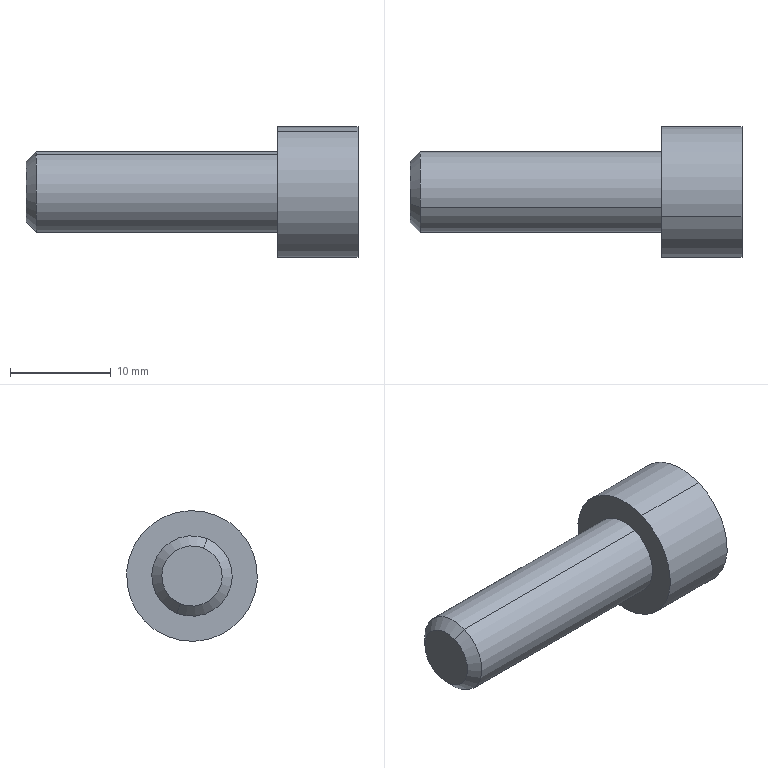Component | SolidWorks | 10HexSocketScrewM8X25-2 | 1 solid | 23 faces | box 33 x 13 x 13 mm | volume 2111 mm3 | plane 15 | cone 4 | cylinder 4 | commonest cylinder face diameters 8 x2 13 x2
STEP:
#1=COLOUR_RGB('',0.7922,0.8196,0.9333);
#2=FILL_AREA_STYLE_COLOUR('',#1);
#3=FILL_AREA_STYLE('',(#2));
#4=SURFACE_STYLE_FILL_AREA(#3);
#5=SURFACE_SIDE_STYLE('',(#4));
#6=SURFACE_STYLE_USAGE(.BOTH.,#5);
#7=PRESENTATION_STYLE_ASSIGNMENT((#6));
#8=CARTESIAN_POINT('',(3.66,-0.8593,8.759));
#9=VERTEX_POINT('',#8);
#10=CARTESIAN_POINT('',(3.66,-0.9495,8.977));
#11=VERTEX_POINT('',#10);
#12=CARTESIAN_POINT('',(3.66,-0.9044,8.868));
#13=DIRECTION('',(-1.,-0.,-0.));
#14=DIRECTION('',(0.,0.3818,-0.9242));
#15=AXIS2_PLACEMENT_3D('',#12,#13,#14);
#16=CIRCLE('',#15,0.1181);
#17=EDGE_CURVE('',#9,#11,#16,.T.);
#18=ORIENTED_EDGE('',*,*,#17,.F.);
#19=CARTESIAN_POINT('',(3.699,-0.8443,8.723));
#20=VERTEX_POINT('',#19);
#21=CARTESIAN_POINT('',(3.66,-0.8593,8.759));
#22=DIRECTION('',(0.7071,0.27,-0.6535));
#23=VECTOR('',#22,39.37);
#24=LINE('',#21,#23);
#25=EDGE_CURVE('',#9,#20,#24,.T.);
#26=ORIENTED_EDGE('',*,*,#25,.T.);
#27=CARTESIAN_POINT('',(3.699,-0.9646,9.014));
#28=VERTEX_POINT('',#27);
#29=CARTESIAN_POINT('',(3.699,-0.9044,8.868));
#30=DIRECTION('',(1.,0.,0.));
#31=DIRECTION('',(0.,0.3818,-0.9242));
#32=AXIS2_PLACEMENT_3D('',#29,#30,#31);
#33=CIRCLE('',#32,0.1575);
#34=EDGE_CURVE('',#28,#20,#33,.T.);
#35=ORIENTED_EDGE('',*,*,#34,.F.);
#36=CARTESIAN_POINT('',(3.66,-0.9495,8.977));
#37=DIRECTION('',(0.7071,-0.27,0.6535));
#38=VECTOR('',#37,39.37);
#39=LINE('',#36,#38);
#40=EDGE_CURVE('',#11,#28,#39,.T.);
#41=ORIENTED_EDGE('',*,*,#40,.F.);
#42=EDGE_LOOP('',(#18,#26,#35,#41));
#43=FACE_OUTER_BOUND('',#42,.T.);
#44=CARTESIAN_POINT('',(3.66,-0.9044,8.868));
#45=DIRECTION('',(1.,0.,0.));
#46=DIRECTION('',(0.,-0.3818,0.9242));
#47=AXIS2_PLACEMENT_3D('',#44,#45,#46);
#48=CONICAL_SURFACE('',#47,0.1181,0.7854);
#49=ADVANCED_FACE('',(#43),#48,.T.);
#50=ORIENTED_EDGE('',*,*,#34,.T.);
#51=CARTESIAN_POINT('',(4.644,-0.8443,8.723));
#52=VERTEX_POINT('',#51);
#53=CARTESIAN_POINT('',(3.66,-0.8443,8.723));
#54=DIRECTION('',(1.,0.,0.));
#55=VECTOR('',#54,39.37);
#56=LINE('',#53,#55);
#57=EDGE_CURVE('',#20,#52,#56,.T.);
#58=ORIENTED_EDGE('',*,*,#57,.T.);
#59=CARTESIAN_POINT('',(4.644,-0.9646,9.014));
#60=VERTEX_POINT('',#59);
#61=CARTESIAN_POINT('',(4.644,-0.9044,8.868));
#62=DIRECTION('',(-1.,-0.,-0.));
#63=DIRECTION('',(0.,0.3818,-0.9242));
#64=AXIS2_PLACEMENT_3D('',#61,#62,#63);
#65=CIRCLE('',#64,0.1575);
#66=EDGE_CURVE('',#52,#60,#65,.T.);
#67=ORIENTED_EDGE('',*,*,#66,.T.);
#68=CARTESIAN_POINT('',(3.66,-0.9646,9.014));
#69=DIRECTION('',(1.,0.,0.));
#70=VECTOR('',#69,39.37);
#71=LINE('',#68,#70);
#72=EDGE_CURVE('',#28,#60,#71,.T.);
#73=ORIENTED_EDGE('',*,*,#72,.F.);
#74=EDGE_LOOP('',(#50,#58,#67,#73));
#75=FACE_OUTER_BOUND('',#74,.T.);
#76=CARTESIAN_POINT('',(3.66,-0.9044,8.868));
#77=DIRECTION('',(1.,0.,0.));
#78=DIRECTION('',(0.,-0.3818,0.9242));
#79=AXIS2_PLACEMENT_3D('',#76,#77,#78);
#80=CYLINDRICAL_SURFACE('',#79,0.1575);
#81=ADVANCED_FACE('',(#75),#80,.T.);
#82=CARTESIAN_POINT('',(4.722,-0.9044,8.868));
#83=VERTEX_POINT('',#82);
#84=CARTESIAN_POINT('',(4.801,-0.9571,8.996));
#85=VERTEX_POINT('',#84);
#86=CARTESIAN_POINT('',(4.801,-0.9571,8.996));
#87=DIRECTION('',(0.5,-0.3307,0.8004));
#88=VECTOR('',#87,39.37);
#89=LINE('',#86,#88);
#90=EDGE_CURVE('',#83,#85,#89,.T.);
#91=ORIENTED_EDGE('',*,*,#90,.F.);
#92=CARTESIAN_POINT('',(4.801,-0.8518,8.741));
#93=VERTEX_POINT('',#92);
#94=CARTESIAN_POINT('',(4.801,-0.8518,8.741));
#95=DIRECTION('',(0.5,0.3307,-0.8004));
#96=VECTOR('',#95,39.37);
#97=LINE('',#94,#96);
#98=EDGE_CURVE('',#83,#93,#97,.T.);
#99=ORIENTED_EDGE('',*,*,#98,.T.);
#100=CARTESIAN_POINT('',(4.801,-0.7952,8.784));
#101=VERTEX_POINT('',#100);
#102=CARTESIAN_POINT('',(4.801,-0.9044,8.868));
#103=DIRECTION('',(1.,0.,0.));
#104=DIRECTION('',(0.,-0.3818,0.9242));
#105=AXIS2_PLACEMENT_3D('',#102,#103,#104);
#106=CIRCLE('',#105,0.1378);
#107=EDGE_CURVE('',#93,#101,#106,.T.);
#108=ORIENTED_EDGE('',*,*,#107,.T.);
#109=CARTESIAN_POINT('',(4.801,-0.7771,8.921));
#110=VERTEX_POINT('',#109);
#111=CARTESIAN_POINT('',(4.801,-0.9044,8.868));
#112=DIRECTION('',(1.,0.,0.));
#113=DIRECTION('',(0.,-0.3818,0.9242));
#114=AXIS2_PLACEMENT_3D('',#111,#112,#113);
#115=CIRCLE('',#114,0.1378);
#116=EDGE_CURVE('',#101,#110,#115,.T.);
#117=ORIENTED_EDGE('',*,*,#116,.T.);
#118=CARTESIAN_POINT('',(4.801,-0.8863,9.005));
#119=VERTEX_POINT('',#118);
#120=CARTESIAN_POINT('',(4.801,-0.9044,8.868));
#121=DIRECTION('',(1.,0.,0.));
#122=DIRECTION('',(0.,-0.3818,0.9242));
#123=AXIS2_PLACEMENT_3D('',#120,#121,#122);
#124=CIRCLE('',#123,0.1378);
#125=EDGE_CURVE('',#110,#119,#124,.T.);
#126=ORIENTED_EDGE('',*,*,#125,.T.);
#127=CARTESIAN_POINT('',(4.801,-0.9044,8.868));
#128=DIRECTION('',(1.,0.,0.));
#129=DIRECTION('',(0.,-0.3818,0.9242));
#130=AXIS2_PLACEMENT_3D('',#127,#128,#129);
#131=CIRCLE('',#130,0.1378);
#132=EDGE_CURVE('',#119,#85,#131,.T.);
#133=ORIENTED_EDGE('',*,*,#132,.T.);
#134=EDGE_LOOP('',(#91,#99,#108,#117,#126,#133));
#135=FACE_OUTER_BOUND('',#134,.T.);
#136=CARTESIAN_POINT('',(4.801,-0.9044,8.868));
#137=DIRECTION('',(1.,0.,0.));
#138=DIRECTION('',(0.,-0.3818,0.9242));
#139=AXIS2_PLACEMENT_3D('',#136,#137,#138);
#140=CONICAL_SURFACE('',#139,0.1378,1.047);
#141=ADVANCED_FACE('',(#135),#140,.F.);
#142=CARTESIAN_POINT('',(4.644,-0.8067,8.632));
#143=VERTEX_POINT('',#142);
#144=CARTESIAN_POINT('',(4.644,-1.002,9.105));
#145=VERTEX_POINT('',#144);
#146=CARTESIAN_POINT('',(4.644,-0.9044,8.868));
#147=DIRECTION('',(-1.,-0.,-0.));
#148=DIRECTION('',(0.,0.3818,-0.9242));
#149=AXIS2_PLACEMENT_3D('',#146,#147,#148);
#150=CIRCLE('',#149,0.2559);
#151=EDGE_CURVE('',#143,#145,#150,.T.);
#152=ORIENTED_EDGE('',*,*,#151,.F.);
#153=CARTESIAN_POINT('',(4.959,-0.8067,8.632));
#154=VERTEX_POINT('',#153);
#155=CARTESIAN_POINT('',(4.644,-0.8067,8.632));
#156=DIRECTION('',(1.,0.,0.));
#157=VECTOR('',#156,39.37);
#158=LINE('',#155,#157);
#159=EDGE_CURVE('',#143,#154,#158,.T.);
#160=ORIENTED_EDGE('',*,*,#159,.T.);
#161=CARTESIAN_POINT('',(4.959,-1.002,9.105));
#162=VERTEX_POINT('',#161);
#163=CARTESIAN_POINT('',(4.959,-0.9044,8.868));
#164=DIRECTION('',(-1.,-0.,-0.));
#165=DIRECTION('',(0.,0.3818,-0.9242));
#166=AXIS2_PLACEMENT_3D('',#163,#164,#165);
#167=CIRCLE('',#166,0.2559);
#168=EDGE_CURVE('',#154,#162,#167,.T.);
#169=ORIENTED_EDGE('',*,*,#168,.T.);
#170=CARTESIAN_POINT('',(4.644,-1.002,9.105));
#171=DIRECTION('',(1.,0.,0.));
#172=VECTOR('',#171,39.37);
#173=LINE('',#170,#172);
#174=EDGE_CURVE('',#145,#162,#173,.T.);
#175=ORIENTED_EDGE('',*,*,#174,.F.);
#176=EDGE_LOOP('',(#152,#160,#169,#175));
#177=FACE_OUTER_BOUND('',#176,.T.);
#178=CARTESIAN_POINT('',(4.644,-0.9044,8.868));
#179=DIRECTION('',(1.,0.,0.));
#180=DIRECTION('',(0.,-0.3818,0.9242));
#181=AXIS2_PLACEMENT_3D('',#178,#179,#180);
#182=CYLINDRICAL_SURFACE('',#181,0.2559);
#183=ADVANCED_FACE('',(#177),#182,.T.);
#184=CARTESIAN_POINT('',(4.801,-1.014,8.952));
#185=VERTEX_POINT('',#184);
#186=CARTESIAN_POINT('',(4.801,-1.032,8.816));
#187=VERTEX_POINT('',#186);
#188=CARTESIAN_POINT('',(4.801,-0.9044,8.868));
#189=DIRECTION('',(1.,0.,0.));
#190=DIRECTION('',(0.,-0.3818,0.9242));
#191=AXIS2_PLACEMENT_3D('',#188,#189,#190);
#192=CIRCLE('',#191,0.1378);
#193=EDGE_CURVE('',#185,#187,#192,.T.);
#194=ORIENTED_EDGE('',*,*,#193,.F.);
#195=CARTESIAN_POINT('',(4.801,-1.062,8.889));
#196=VERTEX_POINT('',#195);
#197=CARTESIAN_POINT('',(4.801,-0.9652,9.015));
#198=DIRECTION('',(0.,-0.6095,-0.7928));
#199=VECTOR('',#198,39.37);
#200=LINE('',#197,#199);
#201=EDGE_CURVE('',#185,#196,#200,.T.);
#202=ORIENTED_EDGE('',*,*,#201,.T.);
#203=CARTESIAN_POINT('',(4.801,-1.062,8.889));
#204=DIRECTION('',(0.,0.3818,-0.9242));
#205=VECTOR('',#204,39.37);
#206=LINE('',#203,#205);
#207=EDGE_CURVE('',#196,#187,#206,.T.);
#208=ORIENTED_EDGE('',*,*,#207,.T.);
#209=EDGE_LOOP('',(#194,#202,#208));
#210=FACE_OUTER_BOUND('',#209,.T.);
#211=CARTESIAN_POINT('',(4.801,-0.9044,8.868));
#212=DIRECTION('',(1.,0.,0.));
#213=DIRECTION('',(-0.,-0.3818,0.9242));
#214=AXIS2_PLACEMENT_3D('',#211,#212,#213);
#215=PLANE('',#214);
#216=ADVANCED_FACE('',(#210),#215,.T.);
#217=CARTESIAN_POINT('',(4.801,-0.9225,8.732));
#218=VERTEX_POINT('',#217);
#219=CARTESIAN_POINT('',(4.801,-0.9044,8.868));
#220=DIRECTION('',(1.,0.,0.));
#221=DIRECTION('',(0.,-0.3818,0.9242));
#222=AXIS2_PLACEMENT_3D('',#219,#220,#221);
#223=CIRCLE('',#222,0.1378);
#224=EDGE_CURVE('',#187,#218,#223,.T.);
#225=ORIENTED_EDGE('',*,*,#224,.F.);
#226=CARTESIAN_POINT('',(4.801,-1.001,8.742));
#227=VERTEX_POINT('',#226);
#228=CARTESIAN_POINT('',(4.801,-1.062,8.889));
#229=DIRECTION('',(0.,0.3818,-0.9242));
#230=VECTOR('',#229,39.37);
#231=LINE('',#228,#230);
#232=EDGE_CURVE('',#187,#227,#231,.T.);
#233=ORIENTED_EDGE('',*,*,#232,.T.);
#234=CARTESIAN_POINT('',(4.801,-1.001,8.742));
#235=DIRECTION('',(0.,0.9913,-0.1314));
#236=VECTOR('',#235,39.37);
#237=LINE('',#234,#236);
#238=EDGE_CURVE('',#227,#218,#237,.T.);
#239=ORIENTED_EDGE('',*,*,#238,.T.);
#240=EDGE_LOOP('',(#225,#233,#239));
#241=FACE_OUTER_BOUND('',#240,.T.);
#242=CARTESIAN_POINT('',(4.801,-0.9044,8.868));
#243=DIRECTION('',(1.,0.,0.));
#244=DIRECTION('',(-0.,-0.3818,0.9242));
#245=AXIS2_PLACEMENT_3D('',#242,#243,#244);
#246=PLANE('',#245);
#247=ADVANCED_FACE('',(#241),#246,.T.);
#248=CARTESIAN_POINT('',(4.801,-0.9044,8.868));
#249=DIRECTION('',(1.,0.,0.));
#250=DIRECTION('',(0.,-0.3818,0.9242));
#251=AXIS2_PLACEMENT_3D('',#248,#249,#250);
#252=CIRCLE('',#251,0.1378);
#253=EDGE_CURVE('',#218,#93,#252,.T.);
#254=ORIENTED_EDGE('',*,*,#253,.F.);
#255=CARTESIAN_POINT('',(4.801,-0.8437,8.721));
#256=VERTEX_POINT('',#255);
#257=CARTESIAN_POINT('',(4.801,-1.001,8.742));
#258=DIRECTION('',(0.,0.9913,-0.1314));
#259=VECTOR('',#258,39.37);
#260=LINE('',#257,#259);
#261=EDGE_CURVE('',#218,#256,#260,.T.);
#262=ORIENTED_EDGE('',*,*,#261,.T.);
#263=CARTESIAN_POINT('',(4.801,-0.8437,8.721));
#264=DIRECTION('',(-0.,0.6095,0.7928));
#265=VECTOR('',#264,39.37);
#266=LINE('',#263,#265);
#267=EDGE_CURVE('',#256,#101,#266,.T.);
#268=ORIENTED_EDGE('',*,*,#267,.T.);
#269=ORIENTED_EDGE('',*,*,#107,.F.);
#270=EDGE_LOOP('',(#254,#262,#268,#269));
#271=FACE_OUTER_BOUND('',#270,.T.);
#272=CARTESIAN_POINT('',(4.801,-0.9044,8.868));
#273=DIRECTION('',(1.,0.,0.));
#274=DIRECTION('',(-0.,-0.3818,0.9242));
#275=AXIS2_PLACEMENT_3D('',#272,#273,#274);
#276=PLANE('',#275);
#277=ADVANCED_FACE('',(#271),#276,.T.);
#278=ORIENTED_EDGE('',*,*,#116,.F.);
#279=CARTESIAN_POINT('',(4.801,-0.7467,8.847));
#280=VERTEX_POINT('',#279);
#281=CARTESIAN_POINT('',(4.801,-0.8437,8.721));
#282=DIRECTION('',(-0.,0.6095,0.7928));
#283=VECTOR('',#282,39.37);
#284=LINE('',#281,#283);
#285=EDGE_CURVE('',#101,#280,#284,.T.);
#286=ORIENTED_EDGE('',*,*,#285,.T.);
#287=CARTESIAN_POINT('',(4.801,-0.7467,8.847));
#288=DIRECTION('',(-0.,-0.3818,0.9242));
#289=VECTOR('',#288,39.37);
#290=LINE('',#287,#289);
#291=EDGE_CURVE('',#280,#110,#290,.T.);
#292=ORIENTED_EDGE('',*,*,#291,.T.);
#293=EDGE_LOOP('',(#278,#286,#292));
#294=FACE_OUTER_BOUND('',#293,.T.);
#295=CARTESIAN_POINT('',(4.801,-0.9044,8.868));
#296=DIRECTION('',(1.,0.,0.));
#297=DIRECTION('',(-0.,-0.3818,0.9242));
#298=AXIS2_PLACEMENT_3D('',#295,#296,#297);
#299=PLANE('',#298);
#300=ADVANCED_FACE('',(#294),#299,.T.);
#301=ORIENTED_EDGE('',*,*,#125,.F.);
#302=CARTESIAN_POINT('',(4.801,-0.8075,8.994));
#303=VERTEX_POINT('',#302);
#304=CARTESIAN_POINT('',(4.801,-0.7467,8.847));
#305=DIRECTION('',(-0.,-0.3818,0.9242));
#306=VECTOR('',#305,39.37);
#307=LINE('',#304,#306);
#308=EDGE_CURVE('',#110,#303,#307,.T.);
#309=ORIENTED_EDGE('',*,*,#308,.T.);
#310=CARTESIAN_POINT('',(4.801,-0.8075,8.994));
#311=DIRECTION('',(-0.,-0.9913,0.1314));
#312=VECTOR('',#311,39.37);
#313=LINE('',#310,#312);
#314=EDGE_CURVE('',#303,#119,#313,.T.);
#315=ORIENTED_EDGE('',*,*,#314,.T.);
#316=EDGE_LOOP('',(#301,#309,#315));
#317=FACE_OUTER_BOUND('',#316,.T.);
#318=CARTESIAN_POINT('',(4.801,-0.9044,8.868));
#319=DIRECTION('',(1.,0.,0.));
#320=DIRECTION('',(-0.,-0.3818,0.9242));
#321=AXIS2_PLACEMENT_3D('',#318,#319,#320);
#322=PLANE('',#321);
#323=ADVANCED_FACE('',(#317),#322,.T.);
#324=ORIENTED_EDGE('',*,*,#159,.F.);
#325=CARTESIAN_POINT('',(4.644,-0.9044,8.868));
#326=DIRECTION('',(-1.,-0.,-0.));
#327=DIRECTION('',(0.,0.3818,-0.9242));
#328=AXIS2_PLACEMENT_3D('',#325,#326,#327);
#329=CIRCLE('',#328,0.2559);
#330=EDGE_CURVE('',#145,#143,#329,.T.);
#331=ORIENTED_EDGE('',*,*,#330,.F.);
#332=ORIENTED_EDGE('',*,*,#174,.T.);
#333=CARTESIAN_POINT('',(4.959,-0.9044,8.868));
#334=DIRECTION('',(-1.,-0.,-0.));
#335=DIRECTION('',(0.,0.3818,-0.9242));
#336=AXIS2_PLACEMENT_3D('',#333,#334,#335);
#337=CIRCLE('',#336,0.2559);
#338=EDGE_CURVE('',#162,#154,#337,.T.);
#339=ORIENTED_EDGE('',*,*,#338,.T.);
#340=EDGE_LOOP('',(#324,#331,#332,#339));
#341=FACE_OUTER_BOUND('',#340,.T.);
#342=CARTESIAN_POINT('',(4.644,-0.9044,8.868));
#343=DIRECTION('',(1.,0.,0.));
#344=DIRECTION('',(0.,-0.3818,0.9242));
#345=AXIS2_PLACEMENT_3D('',#342,#343,#344);
#346=CYLINDRICAL_SURFACE('',#345,0.2559);
#347=ADVANCED_FACE('',(#341),#346,.T.);
#348=CARTESIAN_POINT('',(4.644,-0.9044,8.868));
#349=DIRECTION('',(-1.,-0.,-0.));
#350=DIRECTION('',(0.,0.3818,-0.9242));
#351=AXIS2_PLACEMENT_3D('',#348,#349,#350);
#352=CIRCLE('',#351,0.1575);
#353=EDGE_CURVE('',#60,#52,#352,.T.);
#354=ORIENTED_EDGE('',*,*,#353,.F.);
#355=ORIENTED_EDGE('',*,*,#66,.F.);
#356=EDGE_LOOP('',(#354,#355));
#357=FACE_BOUND('',#356,.T.);
#358=ORIENTED_EDGE('',*,*,#330,.T.);
#359=ORIENTED_EDGE('',*,*,#151,.T.);
#360=EDGE_LOOP('',(#358,#359));
#361=FACE_OUTER_BOUND('',#360,.T.);
#362=CARTESIAN_POINT('',(4.644,-0.9044,8.868));
#363=DIRECTION('',(-1.,-0.,-0.));
#364=DIRECTION('',(0.,0.3818,-0.9242));
#365=AXIS2_PLACEMENT_3D('',#362,#363,#364);
#366=PLANE('',#365);
#367=ADVANCED_FACE('',(#357,#361),#366,.T.);
#368=CARTESIAN_POINT('',(4.959,-0.9652,9.015));
#369=VERTEX_POINT('',#368);
#370=CARTESIAN_POINT('',(4.959,-1.062,8.889));
#371=VERTEX_POINT('',#370);
#372=CARTESIAN_POINT('',(4.959,-0.9652,9.015));
#373=DIRECTION('',(0.,-0.6095,-0.7928));
#374=VECTOR('',#373,39.37);
#375=LINE('',#372,#374);
#376=EDGE_CURVE('',#369,#371,#375,.T.);
#377=ORIENTED_EDGE('',*,*,#376,.F.);
#378=CARTESIAN_POINT('',(4.959,-0.8075,8.994));
#379=VERTEX_POINT('',#378);
#380=CARTESIAN_POINT('',(4.959,-0.8075,8.994));
#381=DIRECTION('',(-0.,-0.9913,0.1314));
#382=VECTOR('',#381,39.37);
#383=LINE('',#380,#382);
#384=EDGE_CURVE('',#379,#369,#383,.T.);
#385=ORIENTED_EDGE('',*,*,#384,.F.);
#386=CARTESIAN_POINT('',(4.959,-0.7467,8.847));
#387=VERTEX_POINT('',#386);
#388=CARTESIAN_POINT('',(4.959,-0.7467,8.847));
#389=DIRECTION('',(-0.,-0.3818,0.9242));
#390=VECTOR('',#389,39.37);
#391=LINE('',#388,#390);
#392=EDGE_CURVE('',#387,#379,#391,.T.);
#393=ORIENTED_EDGE('',*,*,#392,.F.);
#394=CARTESIAN_POINT('',(4.959,-0.8437,8.721));
#395=VERTEX_POINT('',#394);
#396=CARTESIAN_POINT('',(4.959,-0.8437,8.721));
#397=DIRECTION('',(-0.,0.6095,0.7928));
#398=VECTOR('',#397,39.37);
#399=LINE('',#396,#398);
#400=EDGE_CURVE('',#395,#387,#399,.T.);
#401=ORIENTED_EDGE('',*,*,#400,.F.);
#402=CARTESIAN_POINT('',(4.959,-1.001,8.742));
#403=VERTEX_POINT('',#402);
#404=CARTESIAN_POINT('',(4.959,-1.001,8.742));
#405=DIRECTION('',(0.,0.9913,-0.1314));
#406=VECTOR('',#405,39.37);
#407=LINE('',#404,#406);
#408=EDGE_CURVE('',#403,#395,#407,.T.);
#409=ORIENTED_EDGE('',*,*,#408,.F.);
#410=CARTESIAN_POINT('',(4.959,-1.062,8.889));
#411=DIRECTION('',(0.,0.3818,-0.9242));
#412=VECTOR('',#411,39.37);
#413=LINE('',#410,#412);
#414=EDGE_CURVE('',#371,#403,#413,.T.);
#415=ORIENTED_EDGE('',*,*,#414,.F.);
#416=EDGE_LOOP('',(#377,#385,#393,#401,#409,#415));
#417=FACE_BOUND('',#416,.T.);
#418=ORIENTED_EDGE('',*,*,#338,.F.);
#419=ORIENTED_EDGE('',*,*,#168,.F.);
#420=EDGE_LOOP('',(#418,#419));
#421=FACE_OUTER_BOUND('',#420,.T.);
#422=CARTESIAN_POINT('',(4.959,-0.9044,8.868));
#423=DIRECTION('',(-1.,-0.,-0.));
#424=DIRECTION('',(0.,0.3818,-0.9242));
#425=AXIS2_PLACEMENT_3D('',#422,#423,#424);
#426=PLANE('',#425);
#427=ADVANCED_FACE('',(#417,#421),#426,.F.);
#428=ORIENTED_EDGE('',*,*,#384,.T.);
#429=CARTESIAN_POINT('',(4.801,-0.9652,9.015));
#430=VERTEX_POINT('',#429);
#431=CARTESIAN_POINT('',(4.801,-0.9652,9.015));
#432=DIRECTION('',(1.,0.,0.));
#433=VECTOR('',#432,39.37);
#434=LINE('',#431,#433);
#435=EDGE_CURVE('',#430,#369,#434,.T.);
#436=ORIENTED_EDGE('',*,*,#435,.F.);
#437=CARTESIAN_POINT('',(4.801,-0.8075,8.994));
#438=DIRECTION('',(-0.,-0.9913,0.1314));
#439=VECTOR('',#438,39.37);
#440=LINE('',#437,#439);
#441=EDGE_CURVE('',#119,#430,#440,.T.);
#442=ORIENTED_EDGE('',*,*,#441,.F.);
#443=ORIENTED_EDGE('',*,*,#314,.F.);
#444=CARTESIAN_POINT('',(4.801,-0.8075,8.994));
#445=DIRECTION('',(1.,0.,0.));
#446=VECTOR('',#445,39.37);
#447=LINE('',#444,#446);
#448=EDGE_CURVE('',#303,#379,#447,.T.);
#449=ORIENTED_EDGE('',*,*,#448,.T.);
#450=EDGE_LOOP('',(#428,#436,#442,#443,#449));
#451=FACE_OUTER_BOUND('',#450,.T.);
#452=CARTESIAN_POINT('',(4.801,-0.8075,8.994));
#453=DIRECTION('',(-0.,0.1314,0.9913));
#454=DIRECTION('',(0.,0.9913,-0.1314));
#455=AXIS2_PLACEMENT_3D('',#452,#453,#454);
#456=PLANE('',#455);
#457=ADVANCED_FACE('',(#451),#456,.F.);
#458=ORIENTED_EDGE('',*,*,#392,.T.);
#459=ORIENTED_EDGE('',*,*,#448,.F.);
#460=ORIENTED_EDGE('',*,*,#308,.F.);
#461=ORIENTED_EDGE('',*,*,#291,.F.);
#462=CARTESIAN_POINT('',(4.801,-0.7467,8.847));
#463=DIRECTION('',(1.,0.,0.));
#464=VECTOR('',#463,39.37);
#465=LINE('',#462,#464);
#466=EDGE_CURVE('',#280,#387,#465,.T.);
#467=ORIENTED_EDGE('',*,*,#466,.T.);
#468=EDGE_LOOP('',(#458,#459,#460,#461,#467));
#469=FACE_OUTER_BOUND('',#468,.T.);
#470=CARTESIAN_POINT('',(4.801,-0.7467,8.847));
#471=DIRECTION('',(-0.,0.9242,0.3818));
#472=DIRECTION('',(0.,0.3818,-0.9242));
#473=AXIS2_PLACEMENT_3D('',#470,#471,#472);
#474=PLANE('',#473);
#475=ADVANCED_FACE('',(#469),#474,.F.);
#476=ORIENTED_EDGE('',*,*,#400,.T.);
#477=ORIENTED_EDGE('',*,*,#466,.F.);
#478=ORIENTED_EDGE('',*,*,#285,.F.);
#479=ORIENTED_EDGE('',*,*,#267,.F.);
#480=CARTESIAN_POINT('',(4.801,-0.8437,8.721));
#481=DIRECTION('',(1.,0.,0.));
#482=VECTOR('',#481,39.37);
#483=LINE('',#480,#482);
#484=EDGE_CURVE('',#256,#395,#483,.T.);
#485=ORIENTED_EDGE('',*,*,#484,.T.);
#486=EDGE_LOOP('',(#476,#477,#478,#479,#485));
#487=FACE_OUTER_BOUND('',#486,.T.);
#488=CARTESIAN_POINT('',(4.801,-0.8437,8.721));
#489=DIRECTION('',(0.,0.7928,-0.6095));
#490=DIRECTION('',(0.,-0.6095,-0.7928));
#491=AXIS2_PLACEMENT_3D('',#488,#489,#490);
#492=PLANE('',#491);
#493=ADVANCED_FACE('',(#487),#492,.F.);
#494=ORIENTED_EDGE('',*,*,#408,.T.);
#495=ORIENTED_EDGE('',*,*,#484,.F.);
#496=ORIENTED_EDGE('',*,*,#261,.F.);
#497=ORIENTED_EDGE('',*,*,#238,.F.);
#498=CARTESIAN_POINT('',(4.801,-1.001,8.742));
#499=DIRECTION('',(1.,0.,0.));
#500=VECTOR('',#499,39.37);
#501=LINE('',#498,#500);
#502=EDGE_CURVE('',#227,#403,#501,.T.);
#503=ORIENTED_EDGE('',*,*,#502,.T.);
#504=EDGE_LOOP('',(#494,#495,#496,#497,#503));
#505=FACE_OUTER_BOUND('',#504,.T.);
#506=CARTESIAN_POINT('',(4.801,-1.001,8.742));
#507=DIRECTION('',(0.,-0.1314,-0.9913));
#508=DIRECTION('',(-0.,-0.9913,0.1314));
#509=AXIS2_PLACEMENT_3D('',#506,#507,#508);
#510=PLANE('',#509);
#511=ADVANCED_FACE('',(#505),#510,.F.);
#512=ORIENTED_EDGE('',*,*,#414,.T.);
#513=ORIENTED_EDGE('',*,*,#502,.F.);
#514=ORIENTED_EDGE('',*,*,#232,.F.);
#515=ORIENTED_EDGE('',*,*,#207,.F.);
#516=CARTESIAN_POINT('',(4.801,-1.062,8.889));
#517=DIRECTION('',(1.,0.,0.));
#518=VECTOR('',#517,39.37);
#519=LINE('',#516,#518);
#520=EDGE_CURVE('',#196,#371,#519,.T.);
#521=ORIENTED_EDGE('',*,*,#520,.T.);
#522=EDGE_LOOP('',(#512,#513,#514,#515,#521));
#523=FACE_OUTER_BOUND('',#522,.T.);
#524=CARTESIAN_POINT('',(4.801,-1.062,8.889));
#525=DIRECTION('',(0.,-0.9242,-0.3818));
#526=DIRECTION('',(-0.,-0.3818,0.9242));
#527=AXIS2_PLACEMENT_3D('',#524,#525,#526);
#528=PLANE('',#527);
#529=ADVANCED_FACE('',(#523),#528,.F.);
#530=ORIENTED_EDGE('',*,*,#376,.T.);
#531=ORIENTED_EDGE('',*,*,#520,.F.);
#532=ORIENTED_EDGE('',*,*,#201,.F.);
#533=CARTESIAN_POINT('',(4.801,-0.9652,9.015));
#534=DIRECTION('',(0.,-0.6095,-0.7928));
#535=VECTOR('',#534,39.37);
#536=LINE('',#533,#535);
#537=EDGE_CURVE('',#430,#185,#536,.T.);
#538=ORIENTED_EDGE('',*,*,#537,.F.);
#539=ORIENTED_EDGE('',*,*,#435,.T.);
#540=EDGE_LOOP('',(#530,#531,#532,#538,#539));
#541=FACE_OUTER_BOUND('',#540,.T.);
#542=CARTESIAN_POINT('',(4.801,-0.9652,9.015));
#543=DIRECTION('',(-0.,-0.7928,0.6095));
#544=DIRECTION('',(-0.,0.6095,0.7928));
#545=AXIS2_PLACEMENT_3D('',#542,#543,#544);
#546=PLANE('',#545);
#547=ADVANCED_FACE('',(#541),#546,.F.);
#548=ORIENTED_EDGE('',*,*,#132,.F.);
#549=ORIENTED_EDGE('',*,*,#441,.T.);
#550=ORIENTED_EDGE('',*,*,#537,.T.);
#551=CARTESIAN_POINT('',(4.801,-0.9044,8.868));
#552=DIRECTION('',(1.,0.,0.));
#553=DIRECTION('',(0.,-0.3818,0.9242));
#554=AXIS2_PLACEMENT_3D('',#551,#552,#553);
#555=CIRCLE('',#554,0.1378);
#556=EDGE_CURVE('',#85,#185,#555,.T.);
#557=ORIENTED_EDGE('',*,*,#556,.F.);
#558=EDGE_LOOP('',(#548,#549,#550,#557));
#559=FACE_OUTER_BOUND('',#558,.T.);
#560=CARTESIAN_POINT('',(4.801,-0.9044,8.868));
#561=DIRECTION('',(1.,0.,0.));
#562=DIRECTION('',(-0.,-0.3818,0.9242));
#563=AXIS2_PLACEMENT_3D('',#560,#561,#562);
#564=PLANE('',#563);
#565=ADVANCED_FACE('',(#559),#564,.T.);
#566=ORIENTED_EDGE('',*,*,#98,.F.);
#567=ORIENTED_EDGE('',*,*,#90,.T.);
#568=ORIENTED_EDGE('',*,*,#556,.T.);
#569=ORIENTED_EDGE('',*,*,#193,.T.);
#570=ORIENTED_EDGE('',*,*,#224,.T.);
#571=ORIENTED_EDGE('',*,*,#253,.T.);
#572=EDGE_LOOP('',(#566,#567,#568,#569,#570,#571));
#573=FACE_OUTER_BOUND('',#572,.T.);
#574=CARTESIAN_POINT('',(4.801,-0.9044,8.868));
#575=DIRECTION('',(1.,0.,0.));
#576=DIRECTION('',(0.,-0.3818,0.9242));
#577=AXIS2_PLACEMENT_3D('',#574,#575,#576);
#578=CONICAL_SURFACE('',#577,0.1378,1.047);
#579=ADVANCED_FACE('',(#573),#578,.F.);
#580=ORIENTED_EDGE('',*,*,#57,.F.);
#581=CARTESIAN_POINT('',(3.699,-0.9044,8.868));
#582=DIRECTION('',(1.,0.,0.));
#583=DIRECTION('',(0.,0.3818,-0.9242));
#584=AXIS2_PLACEMENT_3D('',#581,#582,#583);
#585=CIRCLE('',#584,0.1575);
#586=EDGE_CURVE('',#20,#28,#585,.T.);
#587=ORIENTED_EDGE('',*,*,#586,.T.);
#588=ORIENTED_EDGE('',*,*,#72,.T.);
#589=ORIENTED_EDGE('',*,*,#353,.T.);
#590=EDGE_LOOP('',(#580,#587,#588,#589));
#591=FACE_OUTER_BOUND('',#590,.T.);
#592=CARTESIAN_POINT('',(3.66,-0.9044,8.868));
#593=DIRECTION('',(1.,0.,0.));
#594=DIRECTION('',(0.,-0.3818,0.9242));
#595=AXIS2_PLACEMENT_3D('',#592,#593,#594);
#596=CYLINDRICAL_SURFACE('',#595,0.1575);
#597=ADVANCED_FACE('',(#591),#596,.T.);
#598=CARTESIAN_POINT('',(3.66,-0.9044,8.868));
#599=DIRECTION('',(-1.,-0.,-0.));
#600=DIRECTION('',(0.,0.3818,-0.9242));
#601=AXIS2_PLACEMENT_3D('',#598,#599,#600);
#602=CIRCLE('',#601,0.1181);
#603=EDGE_CURVE('',#11,#9,#602,.T.);
#604=ORIENTED_EDGE('',*,*,#603,.T.);
#605=ORIENTED_EDGE('',*,*,#17,.T.);
#606=EDGE_LOOP('',(#604,#605));
#607=FACE_OUTER_BOUND('',#606,.T.);
#608=CARTESIAN_POINT('',(3.66,-0.9044,8.868));
#609=DIRECTION('',(-1.,-0.,-0.));
#610=DIRECTION('',(0.,0.3818,-0.9242));
#611=AXIS2_PLACEMENT_3D('',#608,#609,#610);
#612=PLANE('',#611);
#613=ADVANCED_FACE('',(#607),#612,.T.);
#614=ORIENTED_EDGE('',*,*,#25,.F.);
#615=ORIENTED_EDGE('',*,*,#603,.F.);
#616=ORIENTED_EDGE('',*,*,#40,.T.);
#617=ORIENTED_EDGE('',*,*,#586,.F.);
#618=EDGE_LOOP('',(#614,#615,#616,#617));
#619=FACE_OUTER_BOUND('',#618,.T.);
#620=CARTESIAN_POINT('',(3.66,-0.9044,8.868));
#621=DIRECTION('',(1.,0.,0.));
#622=DIRECTION('',(0.,-0.3818,0.9242));
#623=AXIS2_PLACEMENT_3D('',#620,#621,#622);
#624=CONICAL_SURFACE('',#623,0.1181,0.7854);
#625=ADVANCED_FACE('',(#619),#624,.T.);
#626=CLOSED_SHELL('',(#49,#81,#141,#183,#216,#247,#277,#300,#323,#347,#367,#427,#457,#475,#493,#511,#529,#547,#565,#579,#597,#613,#625));
#627=MANIFOLD_SOLID_BREP('',#626);
#628=STYLED_ITEM('',(#7),#627);
#629=(LENGTH_UNIT()NAMED_UNIT(*)SI_UNIT($,.METRE.));
#630=LENGTH_MEASURE_WITH_UNIT(LENGTH_MEASURE(0.0254),#629);
#631=DIMENSIONAL_EXPONENTS(1.,0.,0.,0.,0.,0.,0.);
#632=(CONVERSION_BASED_UNIT('',#630)LENGTH_UNIT()NAMED_UNIT(#631));
#633=UNCERTAINTY_MEASURE_WITH_UNIT(LENGTH_MEASURE(0.00001),#632,'','');
#634=(NAMED_UNIT(*)PLANE_ANGLE_UNIT()SI_UNIT($,.RADIAN.));
#635=(NAMED_UNIT(*)SI_UNIT($,.STERADIAN.)SOLID_ANGLE_UNIT());
#636=(GEOMETRIC_REPRESENTATION_CONTEXT(3)GLOBAL_UNCERTAINTY_ASSIGNED_CONTEXT((#633))GLOBAL_UNIT_ASSIGNED_CONTEXT((#632,#634,#635))REPRESENTATION_CONTEXT('',''));
#637=MECHANICAL_DESIGN_GEOMETRIC_PRESENTATION_REPRESENTATION('',(#628),#636);
#638=PRESENTATION_LAYER_ASSIGNMENT('','',(#628));
#639=CARTESIAN_POINT('',(0.,0.,0.));
#640=DIRECTION('',(0.,0.,1.));
#641=DIRECTION('',(1.,0.,0.));
#642=AXIS2_PLACEMENT_3D('',#639,#640,#641);
#643=(LENGTH_UNIT()NAMED_UNIT(*)SI_UNIT($,.METRE.));
#644=LENGTH_MEASURE_WITH_UNIT(LENGTH_MEASURE(0.0254),#643);
#645=DIMENSIONAL_EXPONENTS(1.,0.,0.,0.,0.,0.,0.);
#646=(CONVERSION_BASED_UNIT('',#644)LENGTH_UNIT()NAMED_UNIT(#645));
#647=UNCERTAINTY_MEASURE_WITH_UNIT(LENGTH_MEASURE(0.00001),#646,'','');
#648=(NAMED_UNIT(*)PLANE_ANGLE_UNIT()SI_UNIT($,.RADIAN.));
#649=(NAMED_UNIT(*)SI_UNIT($,.STERADIAN.)SOLID_ANGLE_UNIT());
#650=(GEOMETRIC_REPRESENTATION_CONTEXT(3)GLOBAL_UNCERTAINTY_ASSIGNED_CONTEXT((#647))GLOBAL_UNIT_ASSIGNED_CONTEXT((#646,#648,#649))REPRESENTATION_CONTEXT('',''));
#651=ADVANCED_BREP_SHAPE_REPRESENTATION('',(#627,#642),#650);